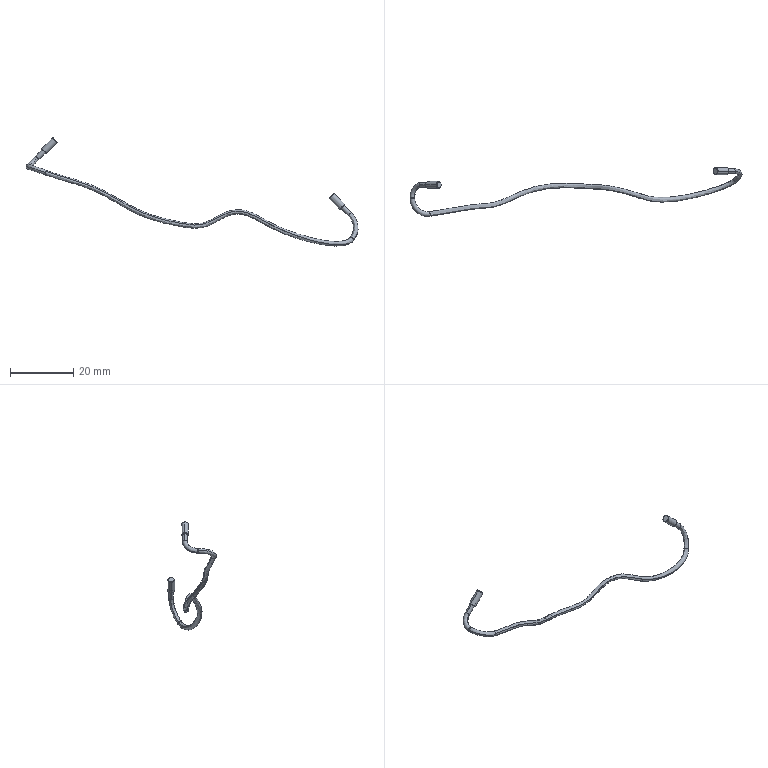Component | SolidWorks | Crijevo_paX4-1 | 3 solids | 56 faces | box 105.41 x 15.49 x 34.35 mm | volume 95 mm3 | cylinder 20 | torus 16 | plane 8 | spline 8 | cone 4 | commonest cylinder face diameters 1.5 x10 1.3 x6 2.2 x4